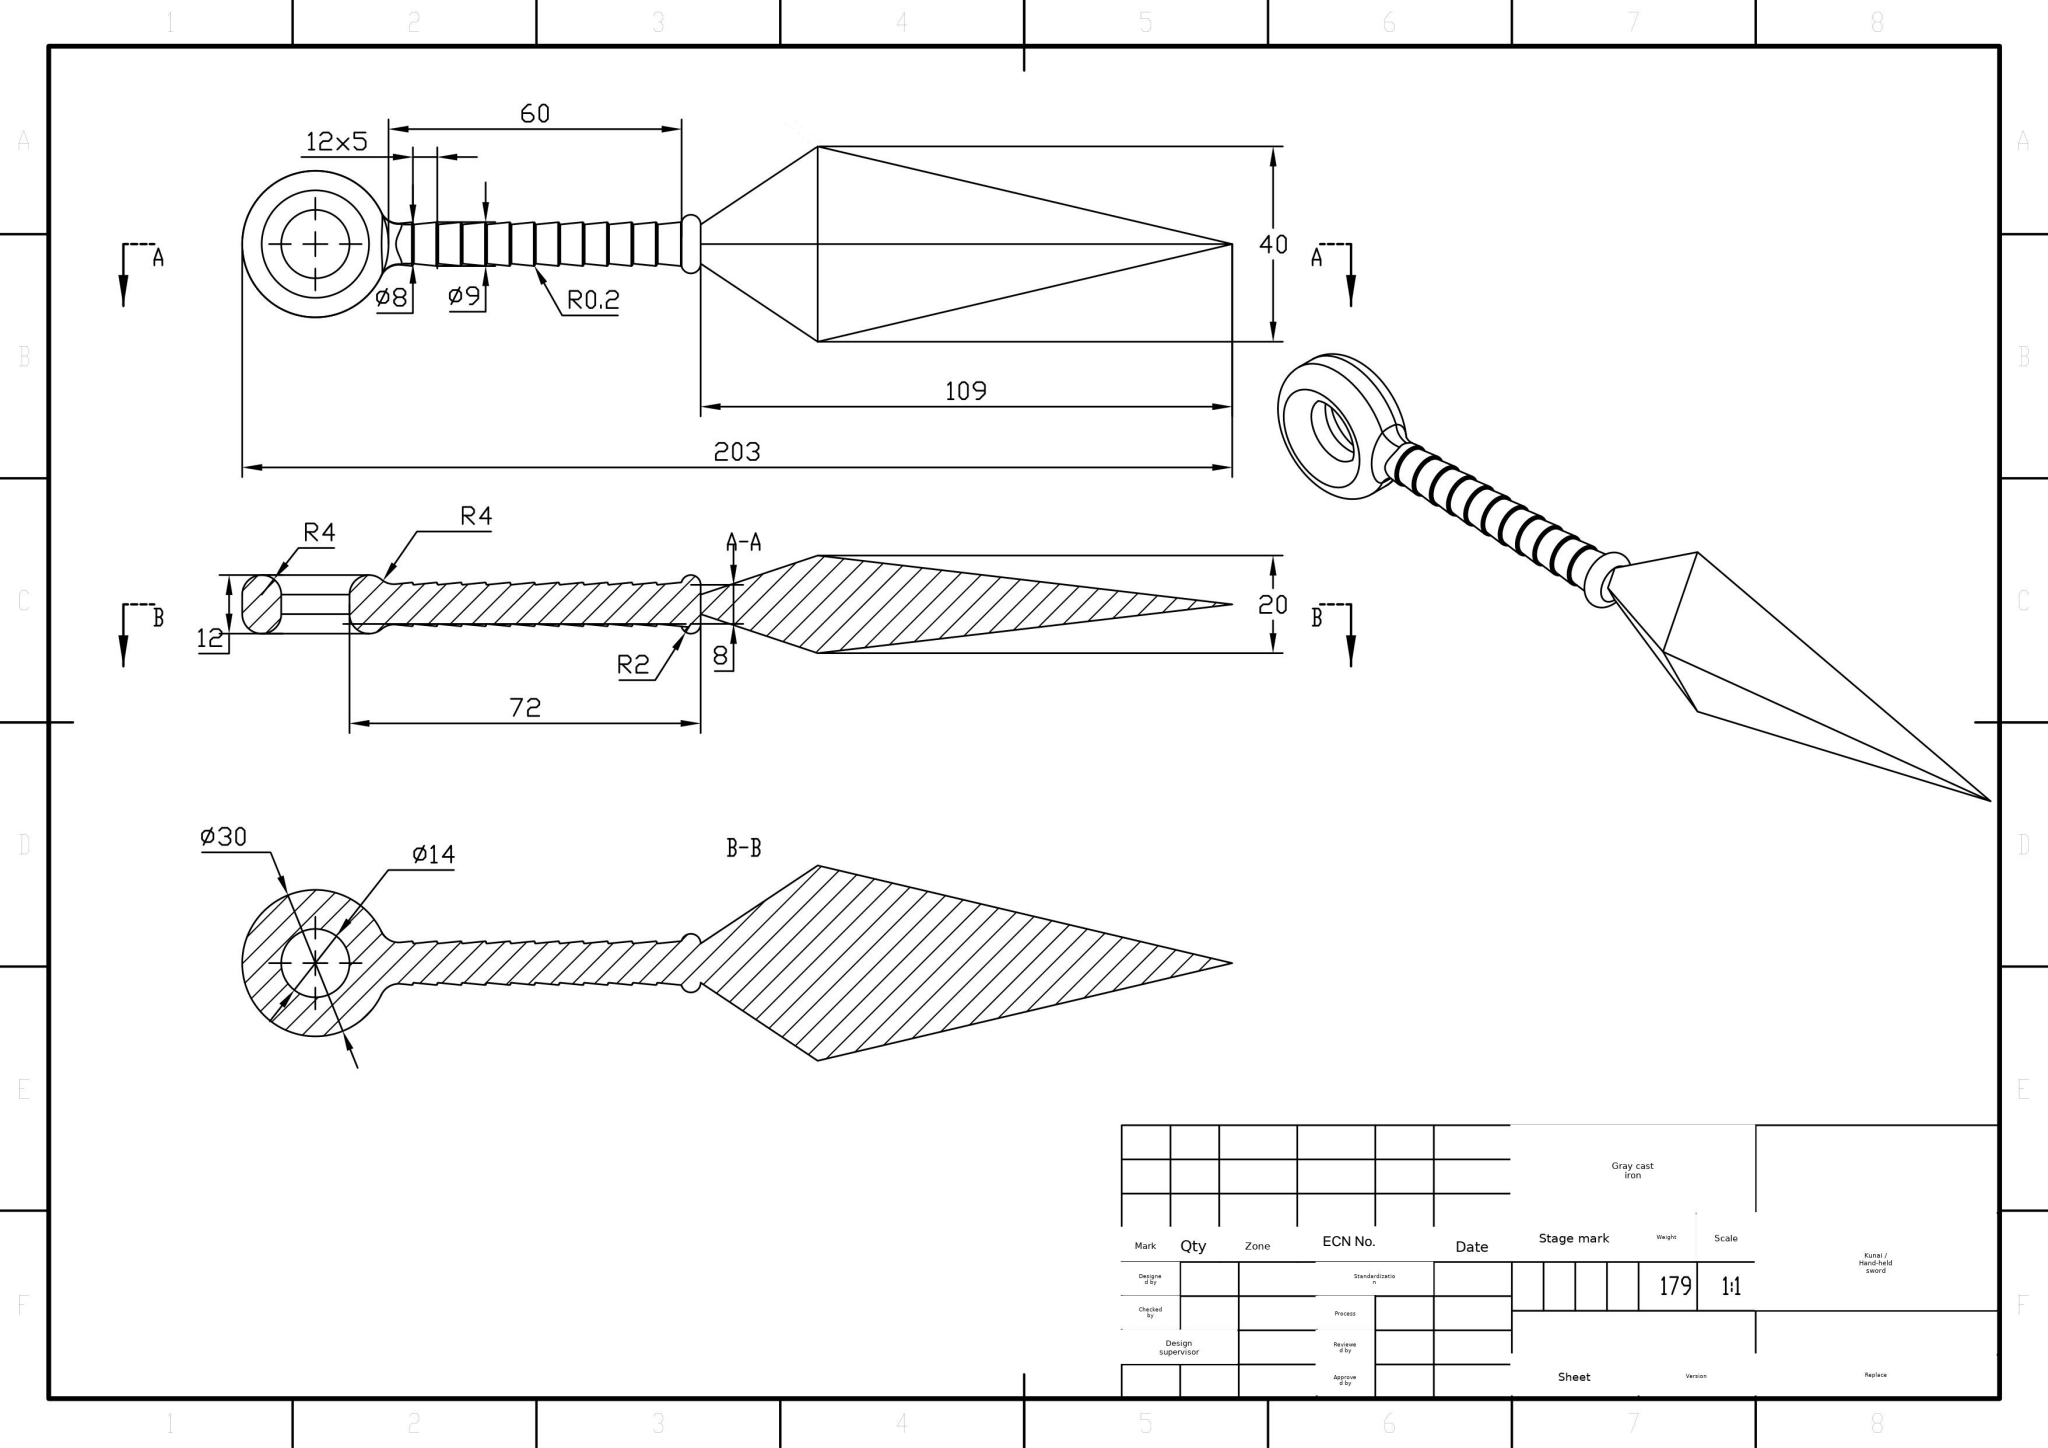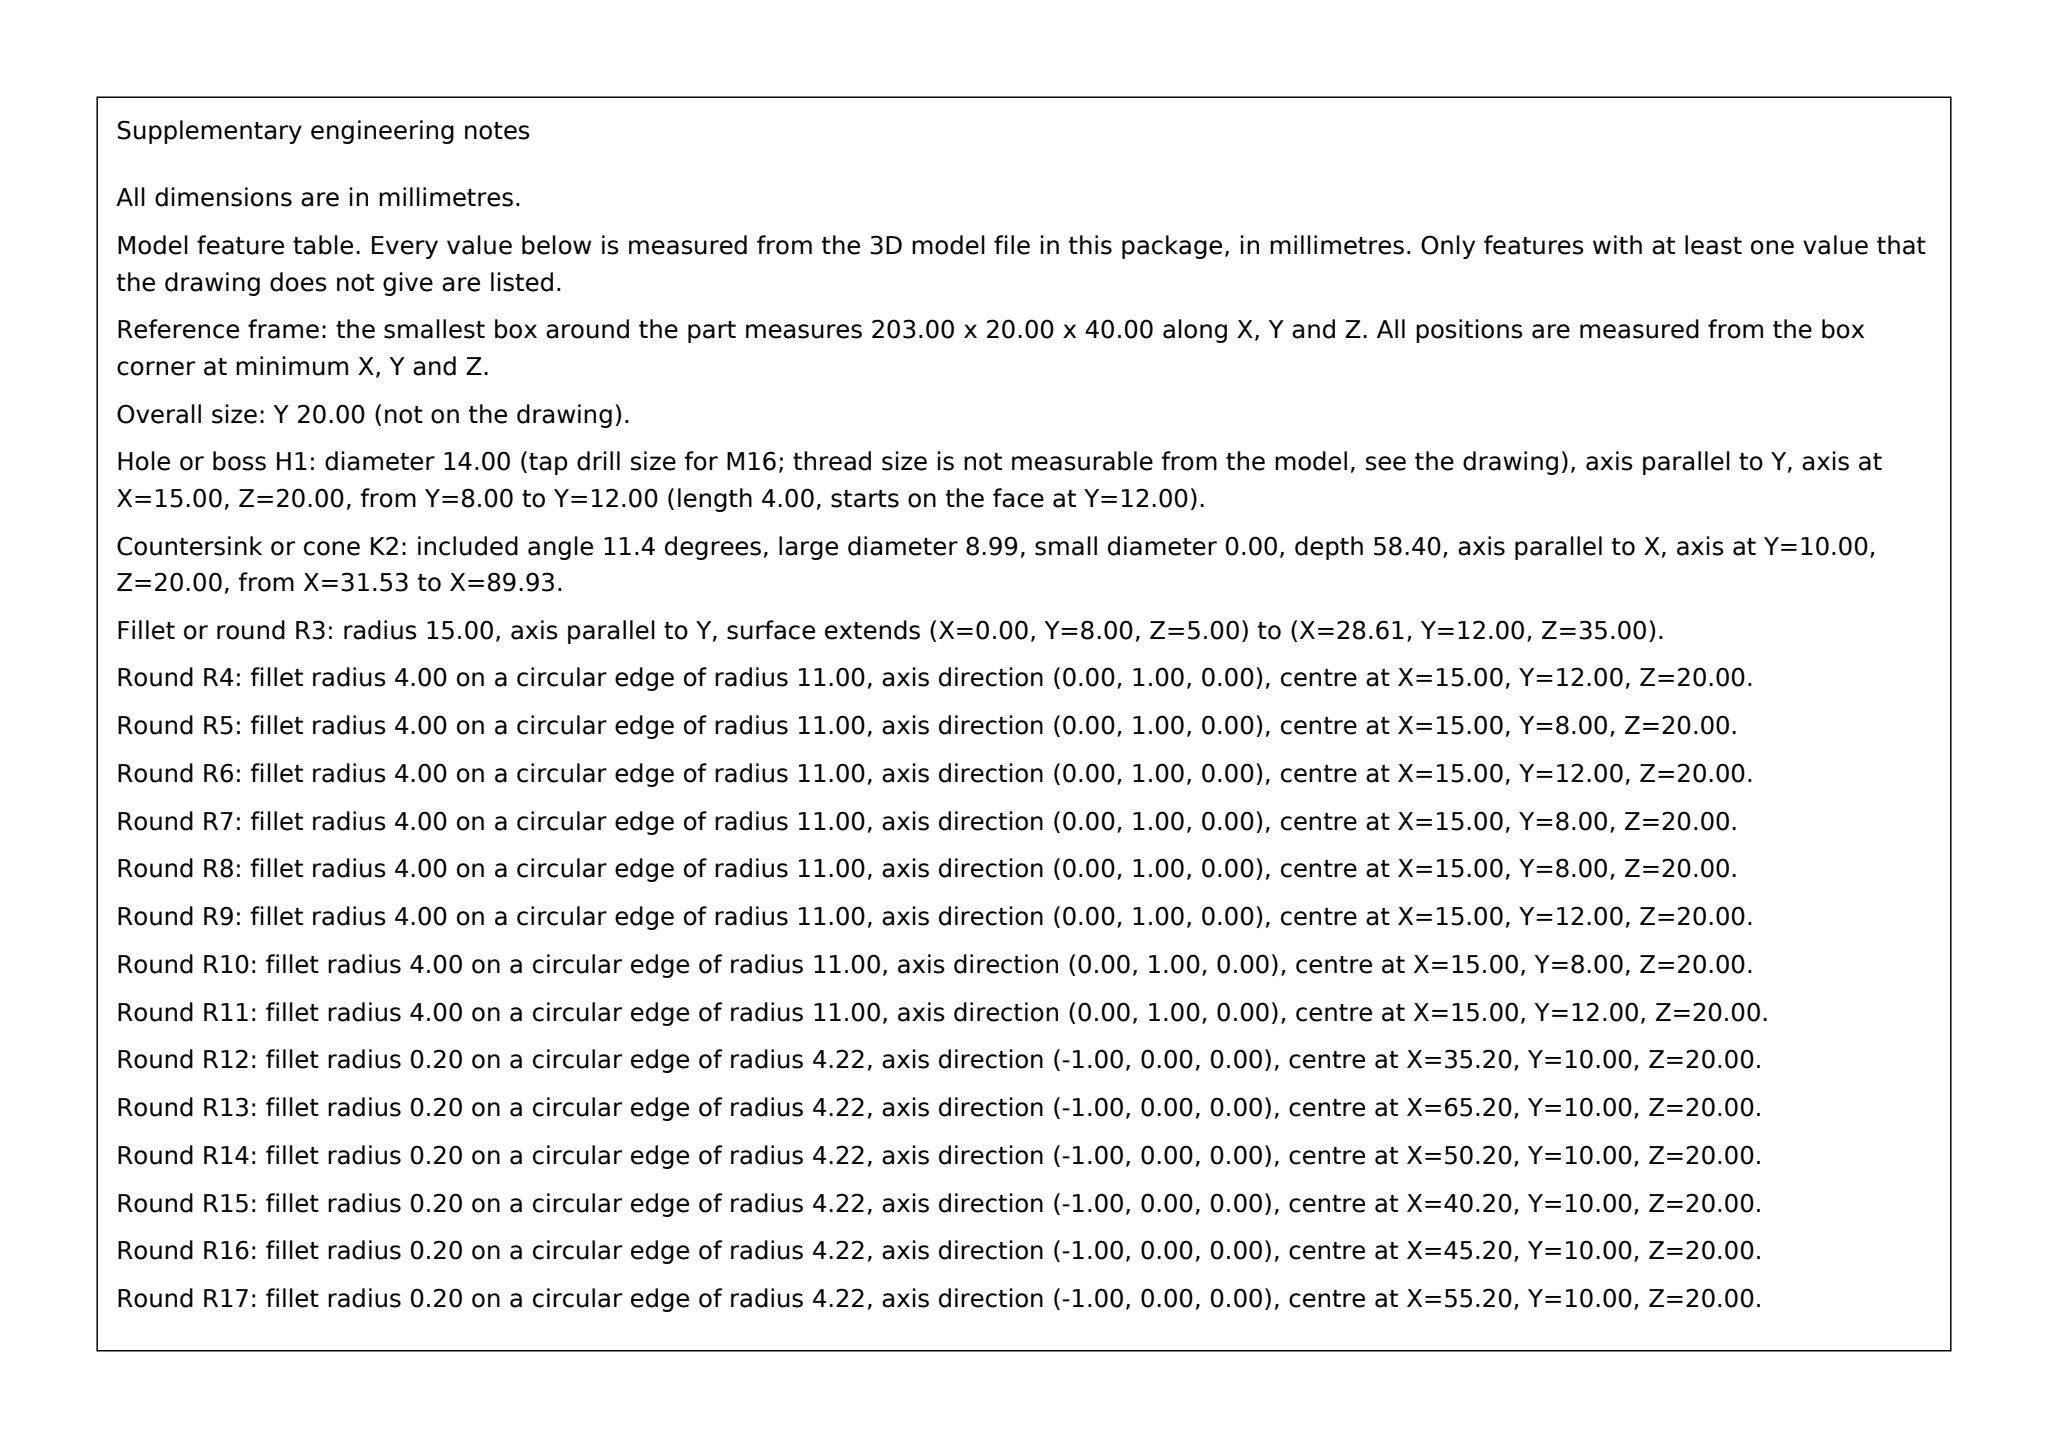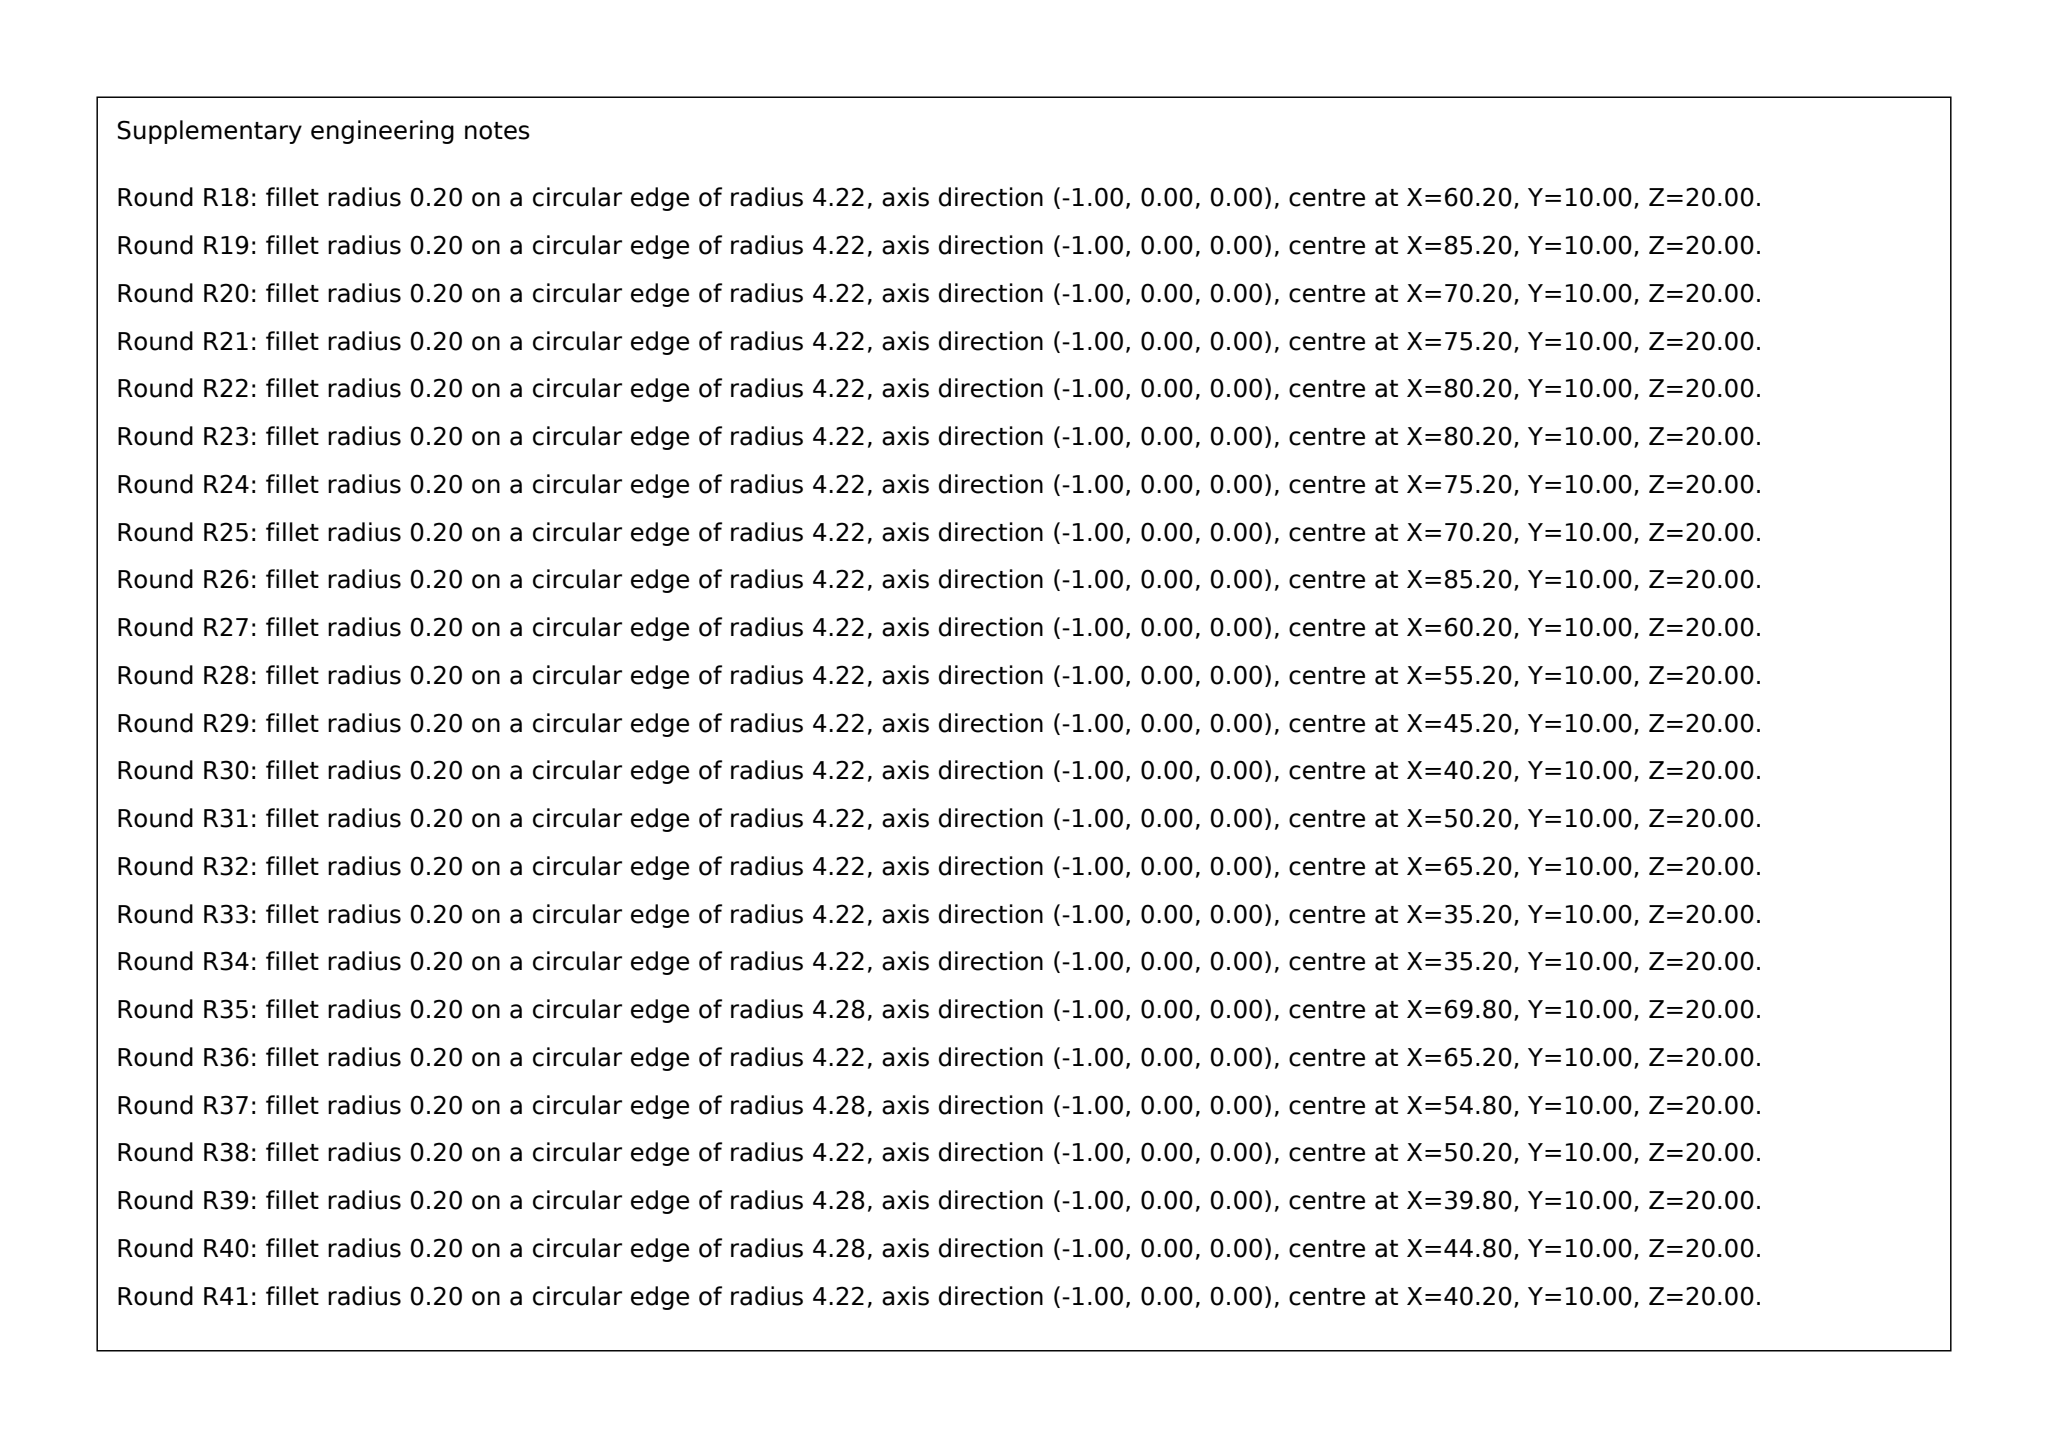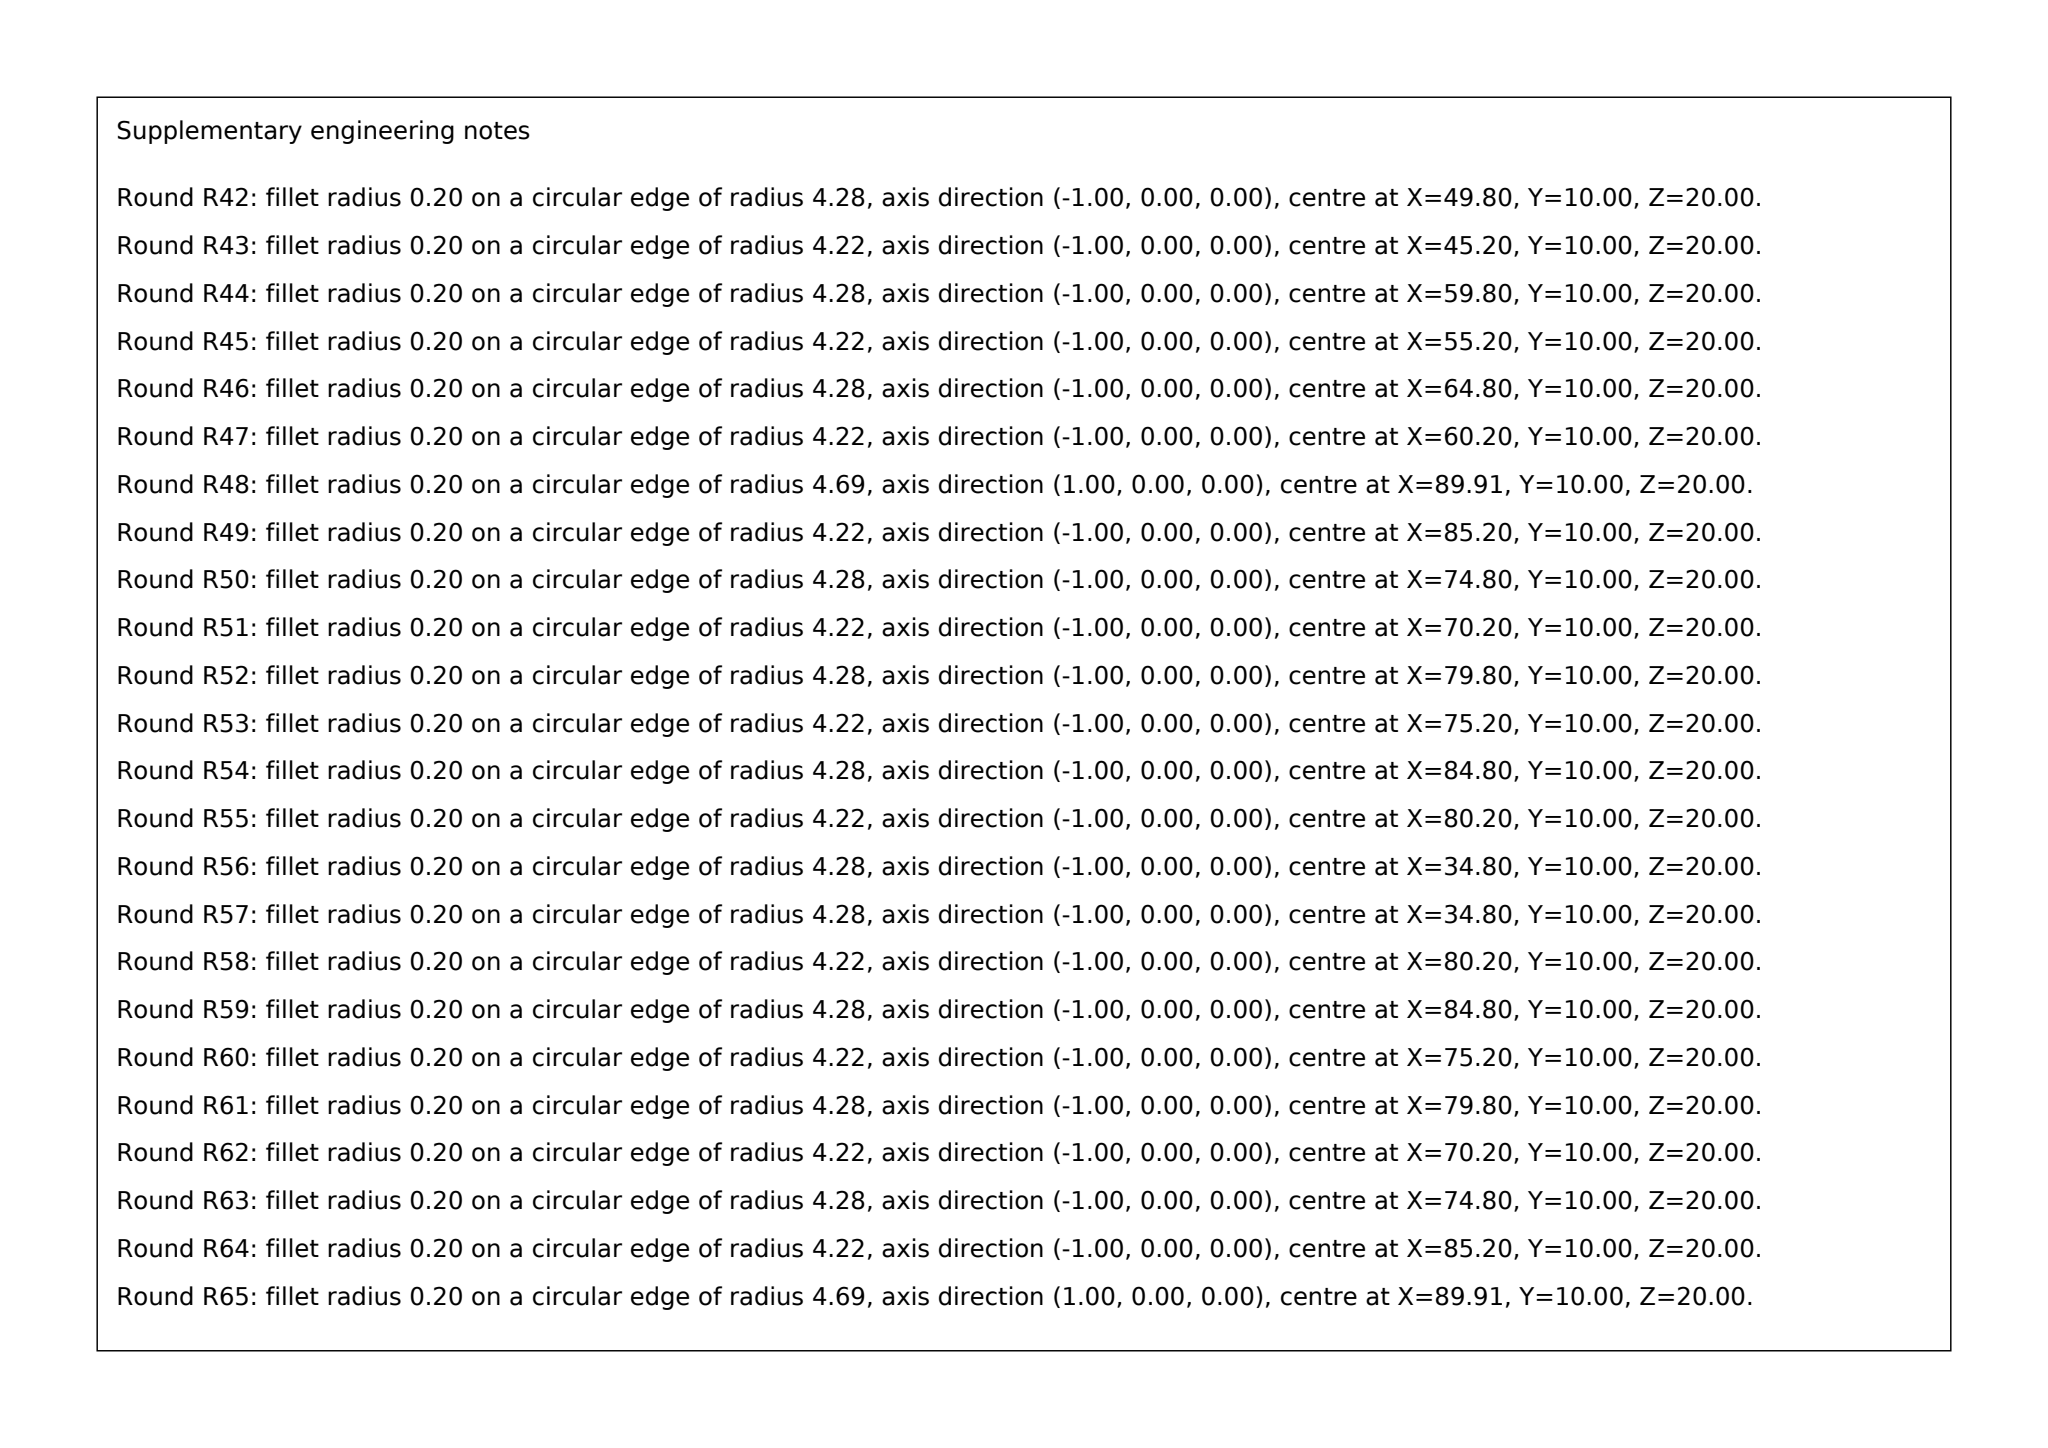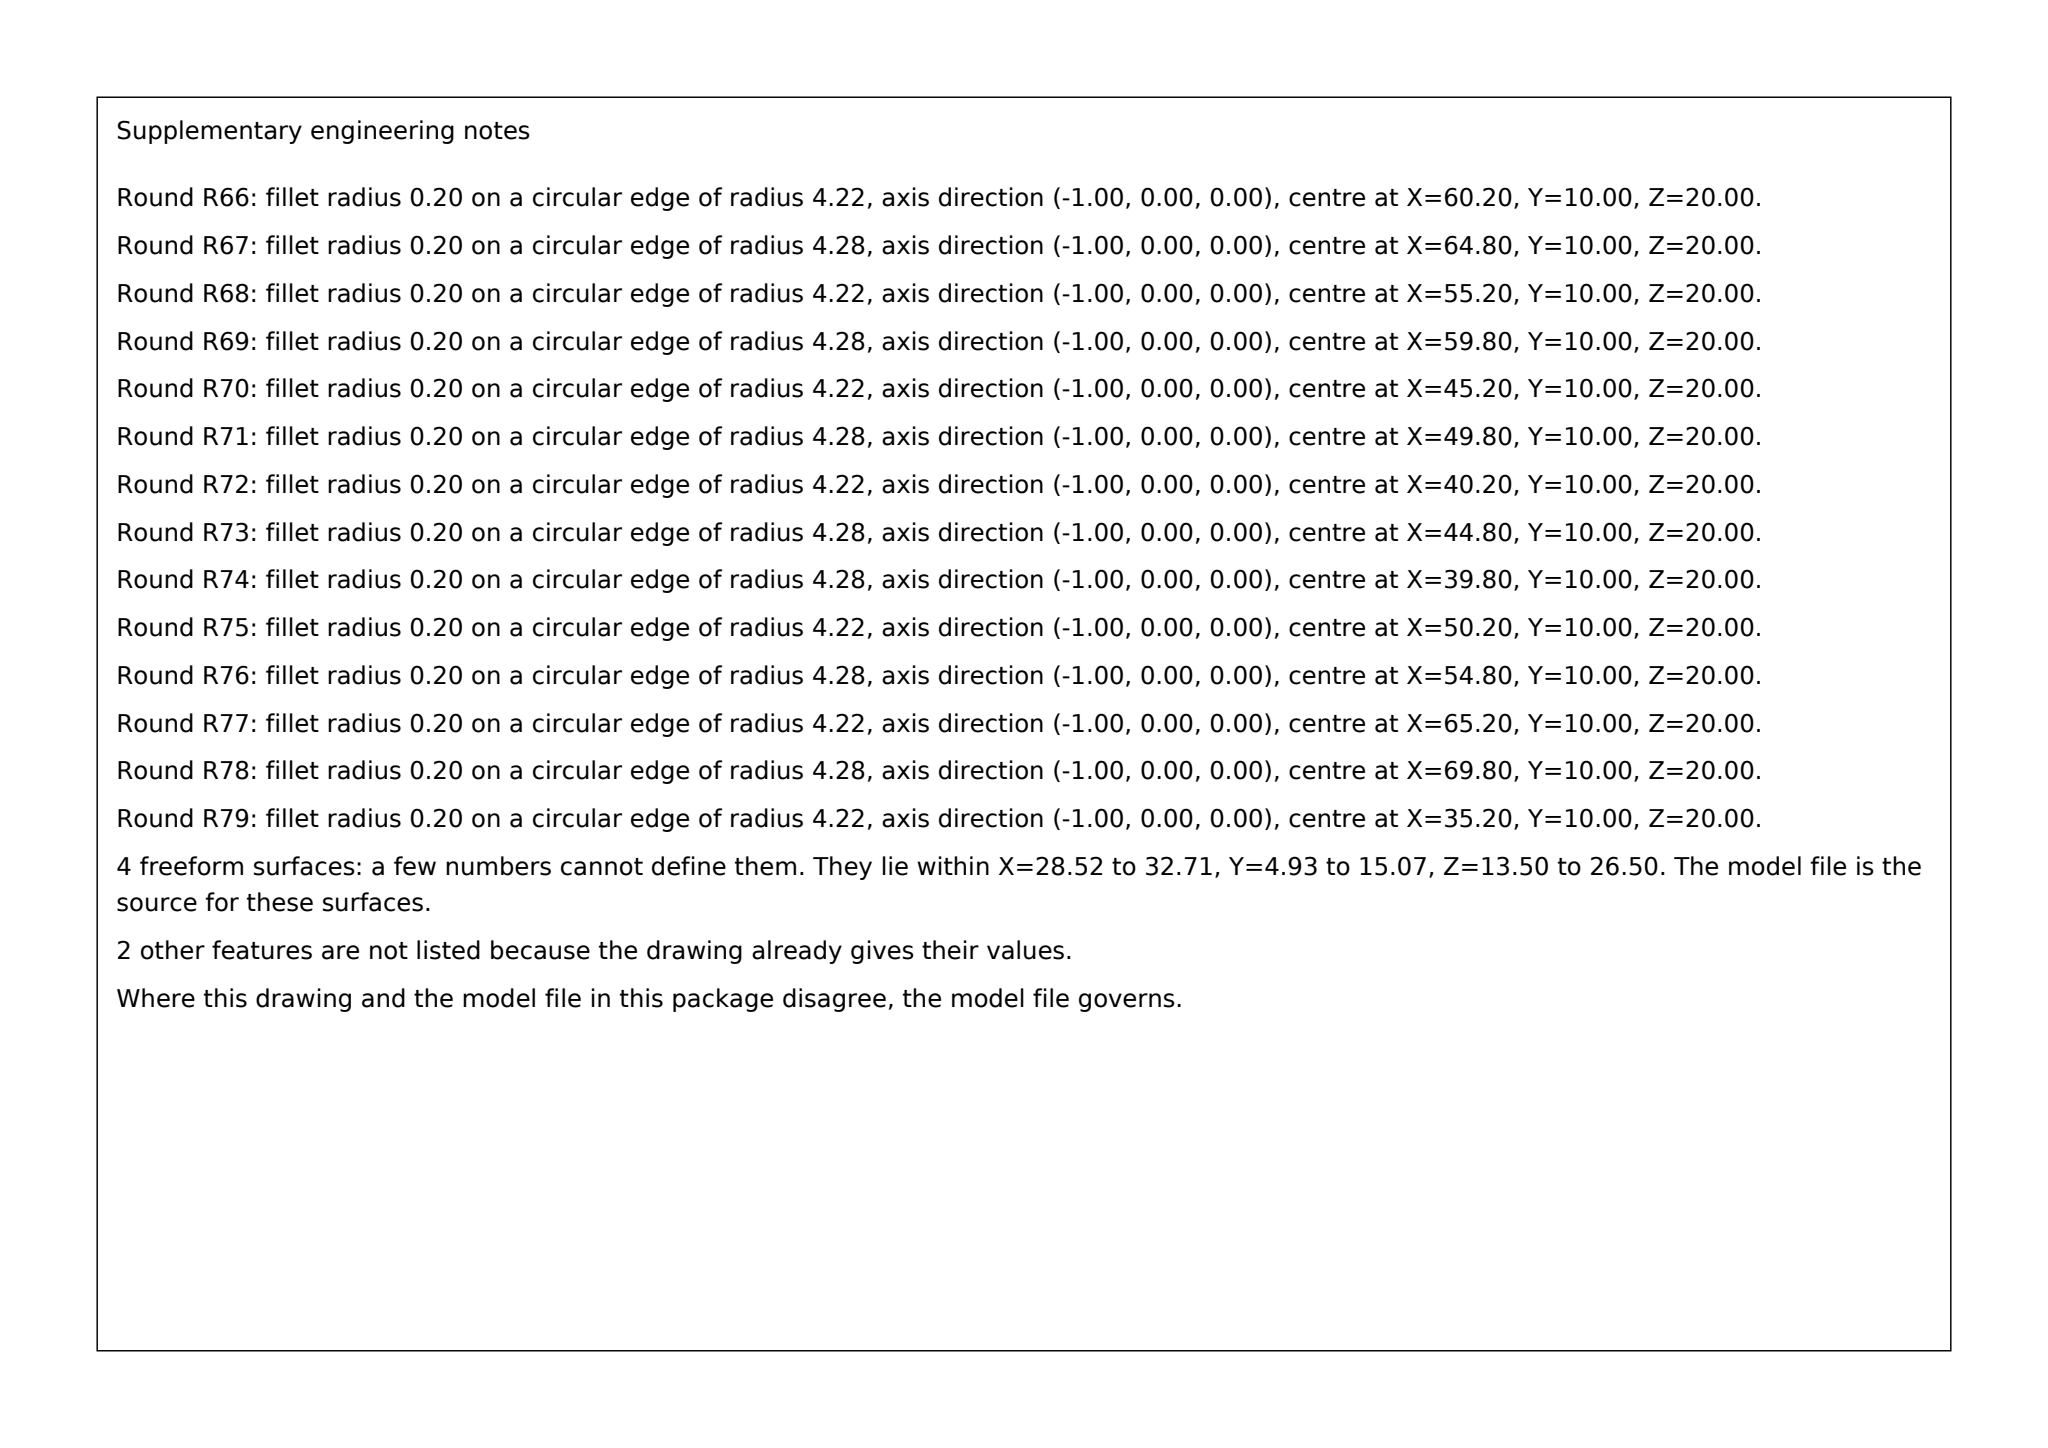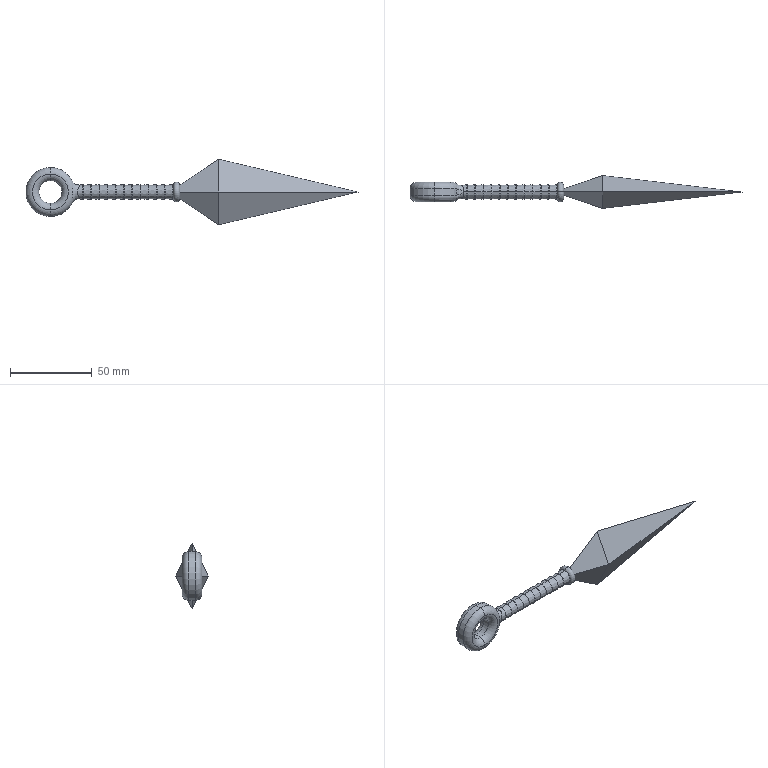Part | SolidWorks | mm | material Gray cast iron | 1 solid | 132 faces | box 203 x 20 x 40 mm | volume 24831 mm3 | torus 78 | cone 24 | plane 21 | cylinder 5 | spline 4 | commonest cylinder face diameters 30 x3 14 x2